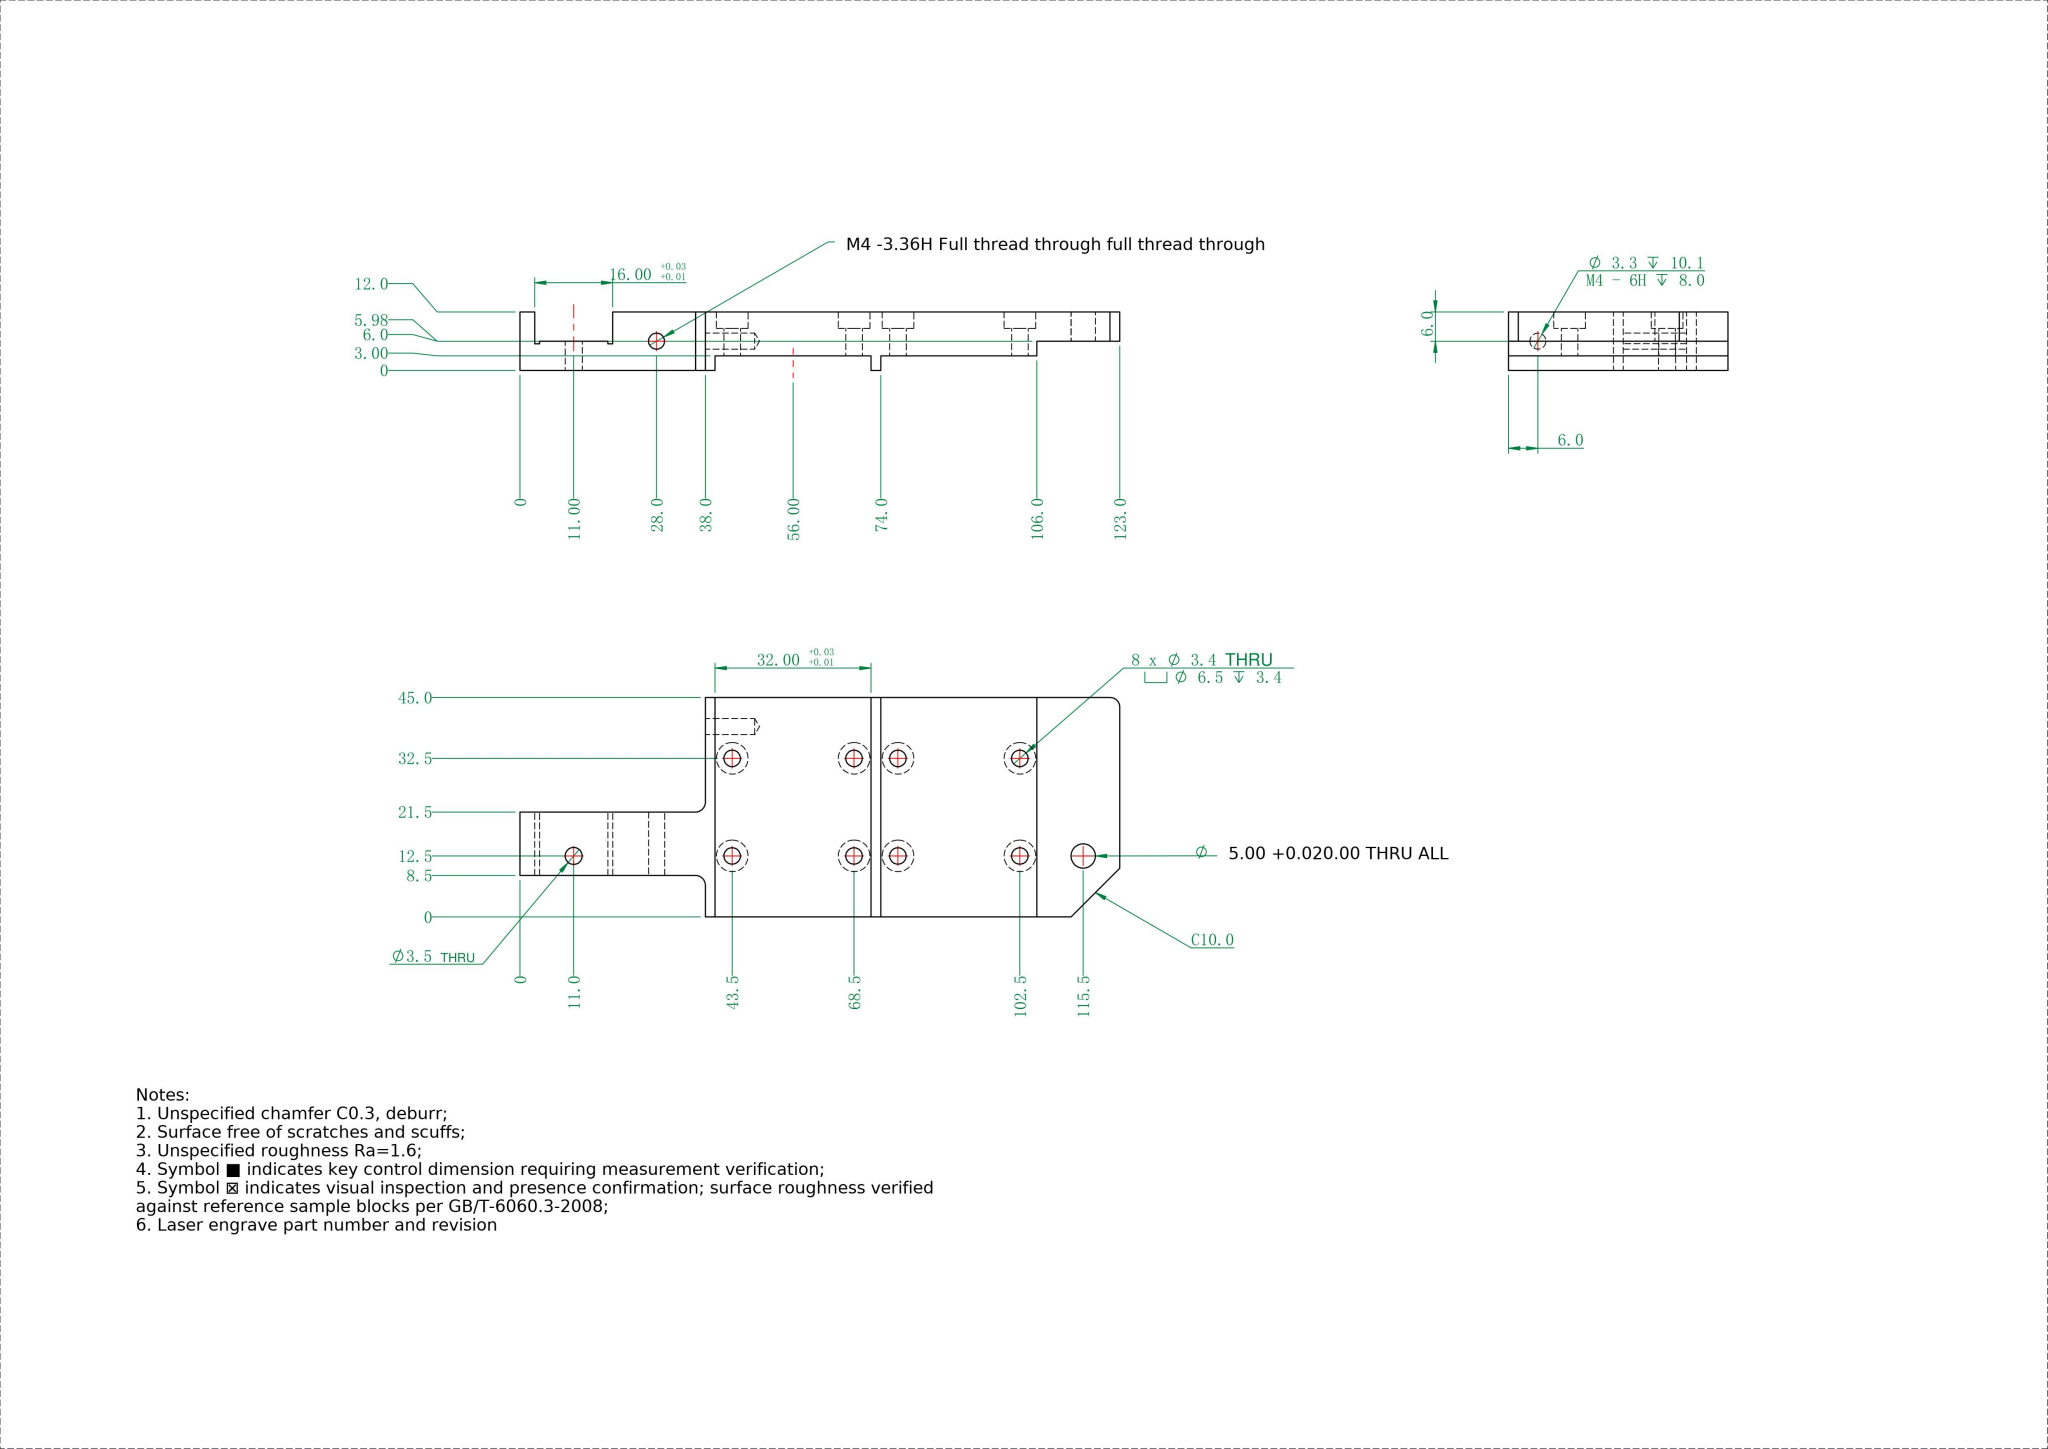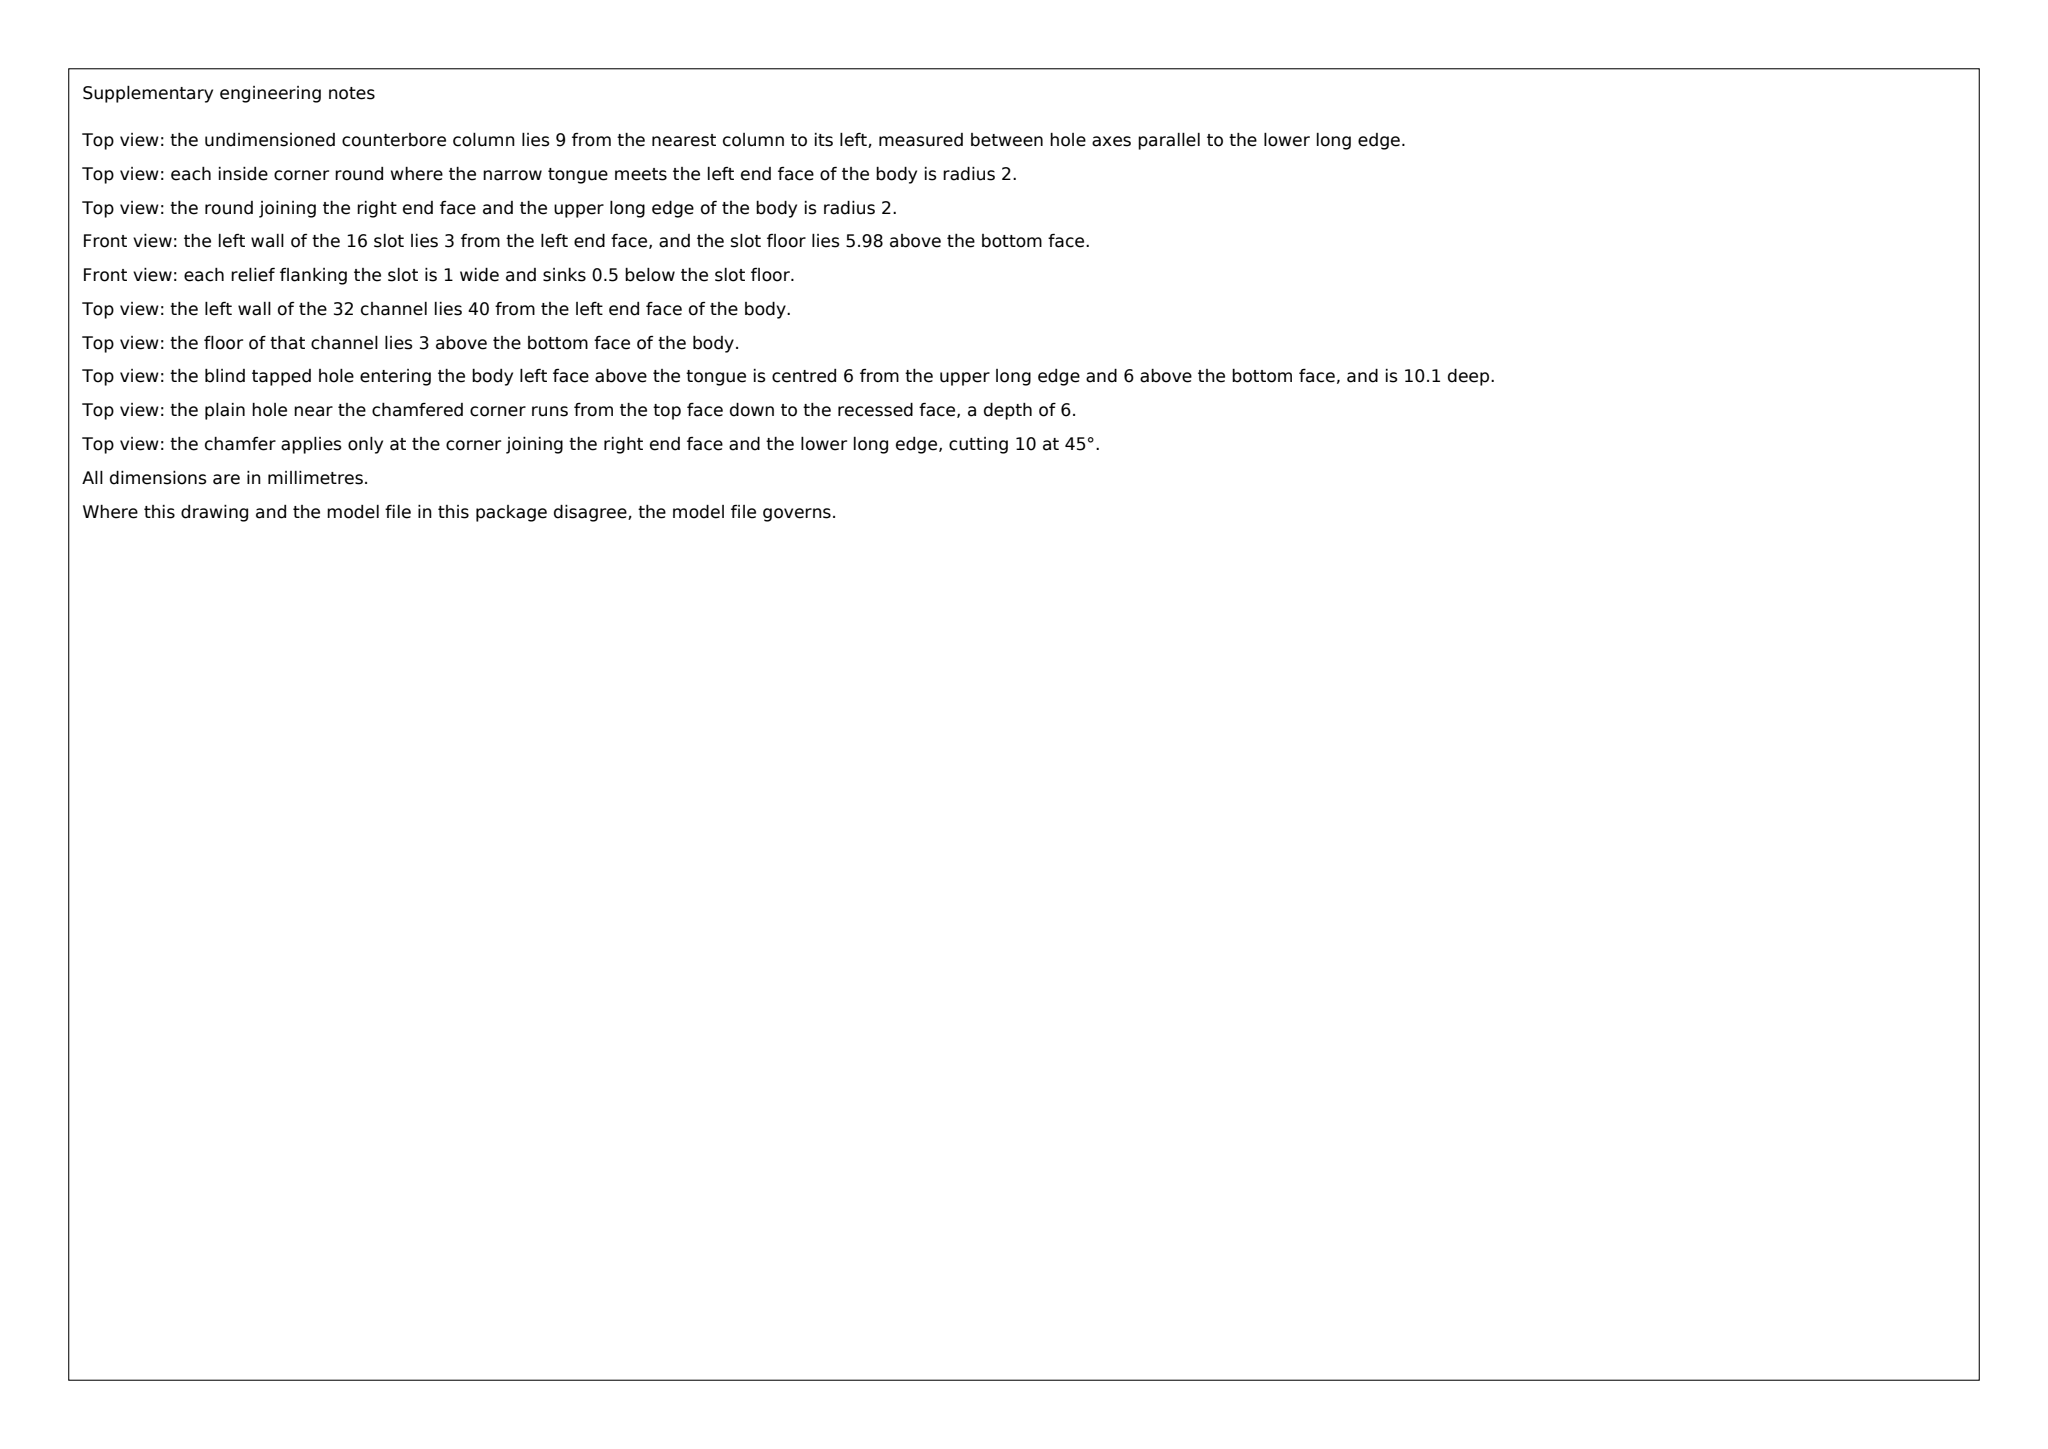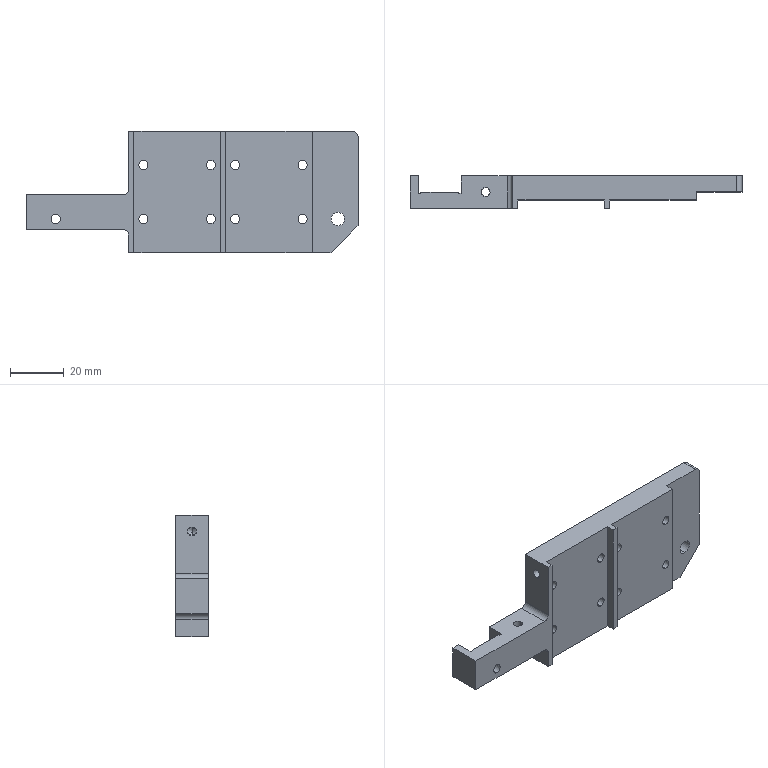Part | SolidWorks | mm | 1 solid | 80 faces | box 123 x 12 x 45 mm | volume 35363 mm3 | cylinder 43 | plane 35 | cone 2 | commonest cylinder face diameters 6.5 x16 3.4 x16 3.3 x4 4 x3 3.5 x2 5 x2
Drawing notes:
OVERALL 123.0 x 45.0 x 12.0 THK | from the solid: bbox_xyz [123.0, 12.0, 45.0]
U/SIDE RECESS X40.0-106.0 x 3.0 DP, FULL WIDTH; RIB X72.0-74.0 | from the solid: x-planes 40,72,74,106; y-planes 0 (rib btm) and 3.0 (recess btm); no z-plane split -> full width
2X 1.0 WIDE GROOVE AT X3.0-4.0 & X18.0-19.0, 0.5 DP FROM 5.98 FACE | from the solid: x-planes 3/4 and 18/19 (1.0 wide); y-plane 5.48 vs flange top 5.98 -> 0.50 deep
M4 AT X28.0, Y6.0 THRU 13.0 VERT (FLANGE Z8.5-21.5) | from the solid: cylinder [3.3, axis z, x=28.0, y=6.0, length 13.0] through flange z 8.5-21.5
SIDE Ø3.3 DP 10.1 FROM X38.0 FACE AT Y6.0, Z39.0; M4-6H DP 8.0 | from the solid: cylinder [3.3, axis x, pos y=6.0 z=39.0, length 10.1] starting at x-plane 38.0; M4-6H ↧8.0 callout
Ø4.0 THRU: 36.0 FROM LH EDGE, 6.5 FROM BTM EDGE | from the solid: cylinder dia 4.0 axis y at [36.0,null,6.5], length 12.0 = full thickness
Ø4.0 THRU: 36.0 FROM LH EDGE, 23.5 FROM BTM EDGE | from the solid: cylinder dia 4.0 axis y at [36.0,null,23.5], length 12.0 = full thickness
Ø4.0 DP 6.0: 121.0 FROM LH EDGE, 43.0 FROM BTM EDGE | from the solid: cylinder dia 4.0 axis y at [121.0,null,43.0], length 6.0 in 12.0 thk = blind